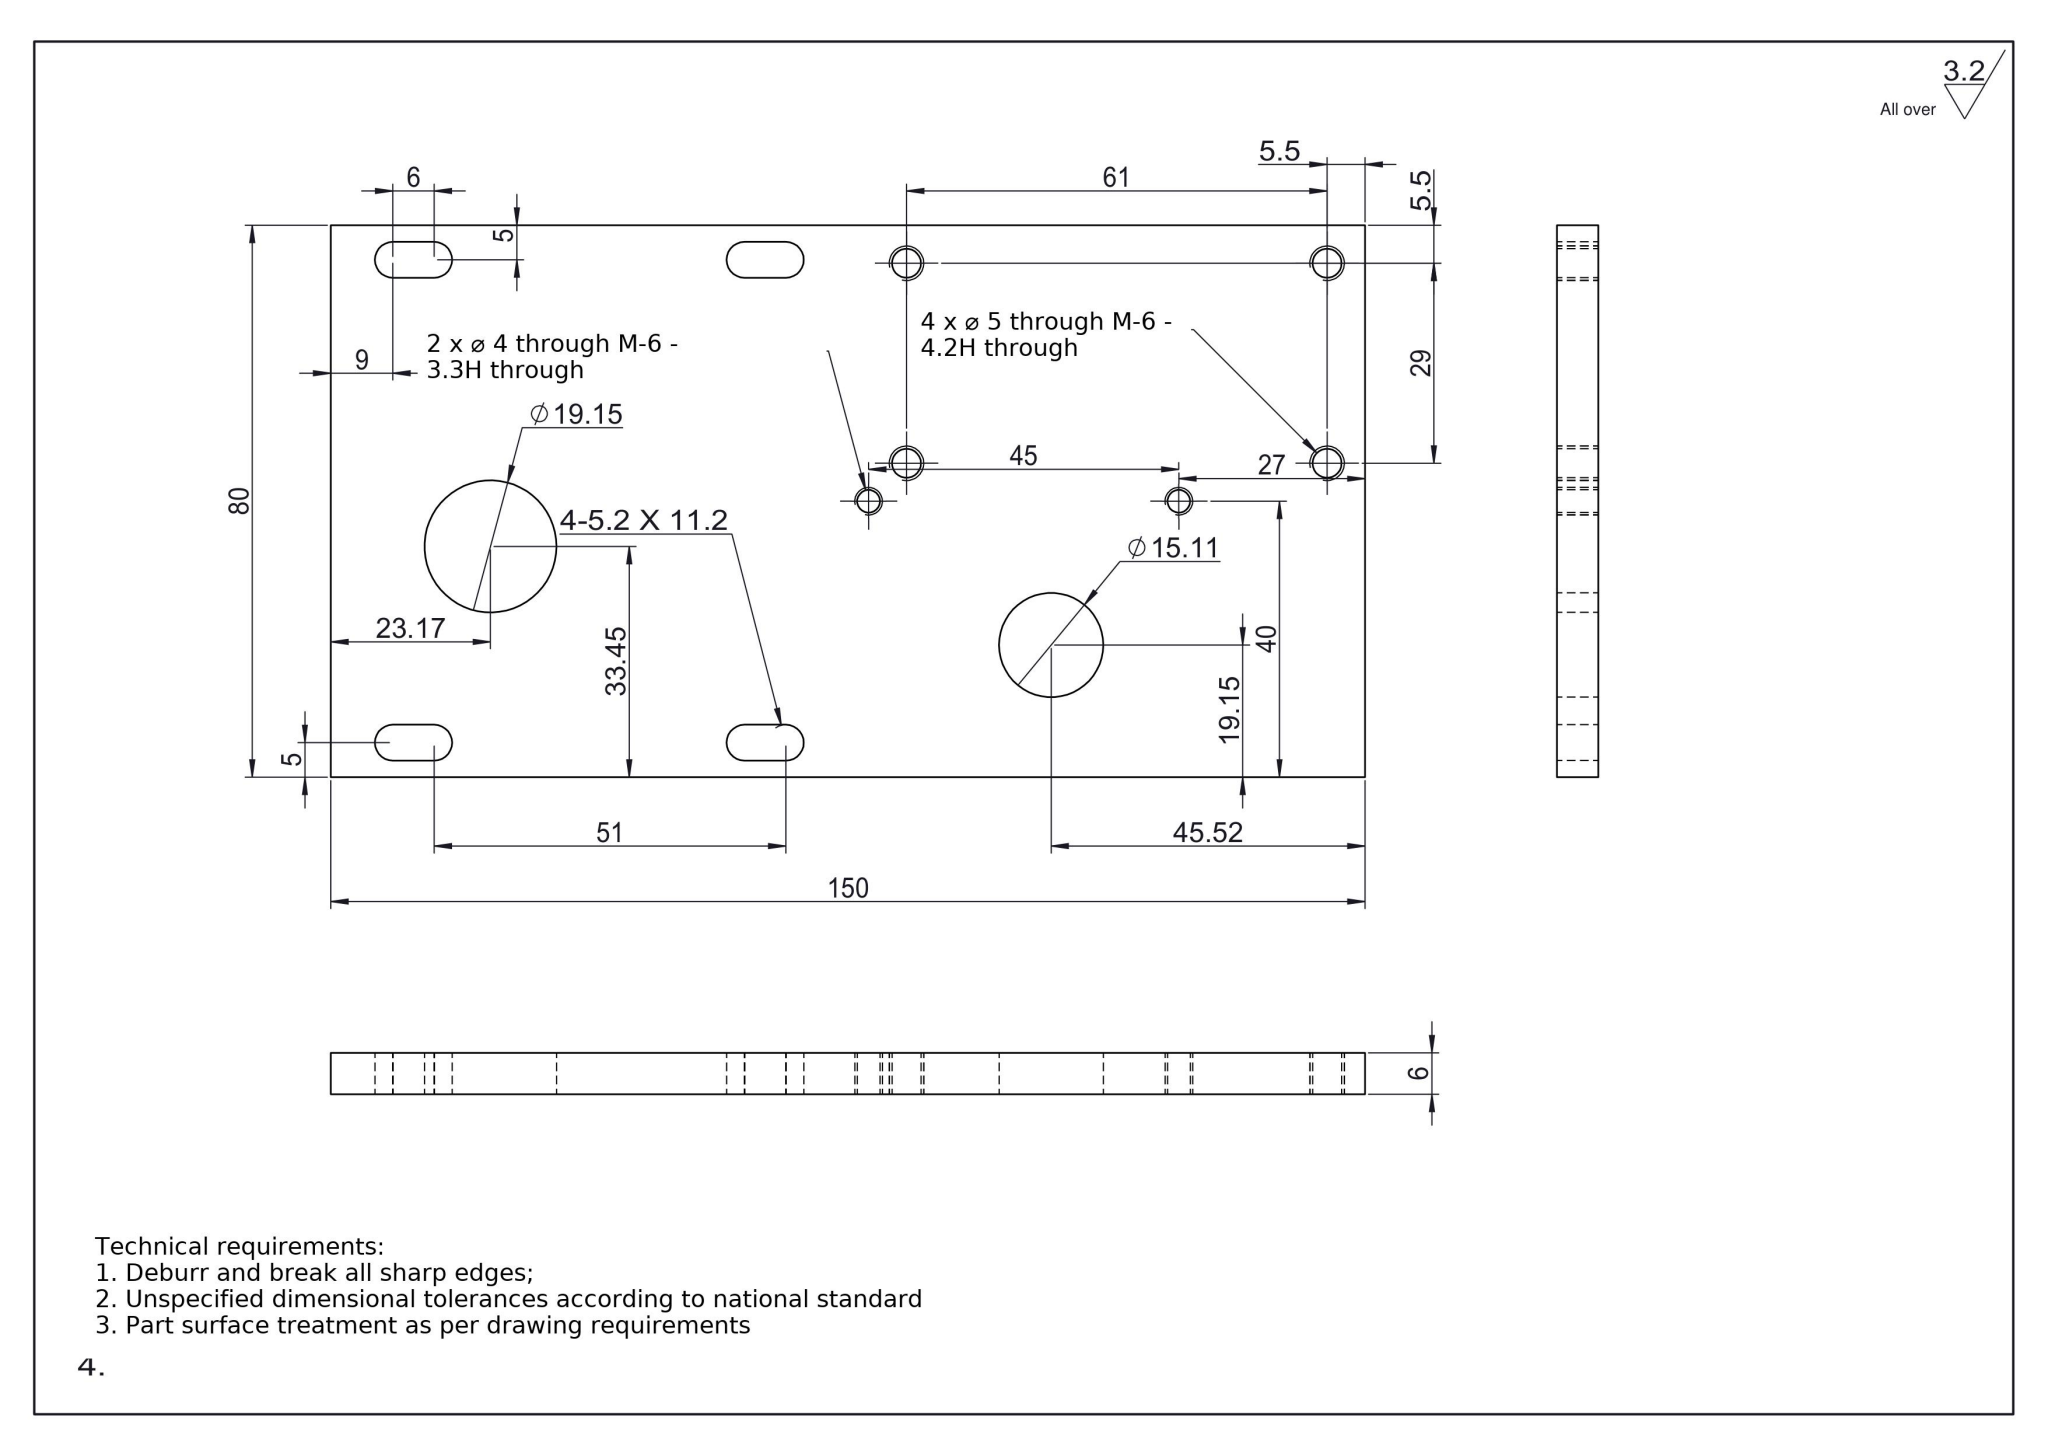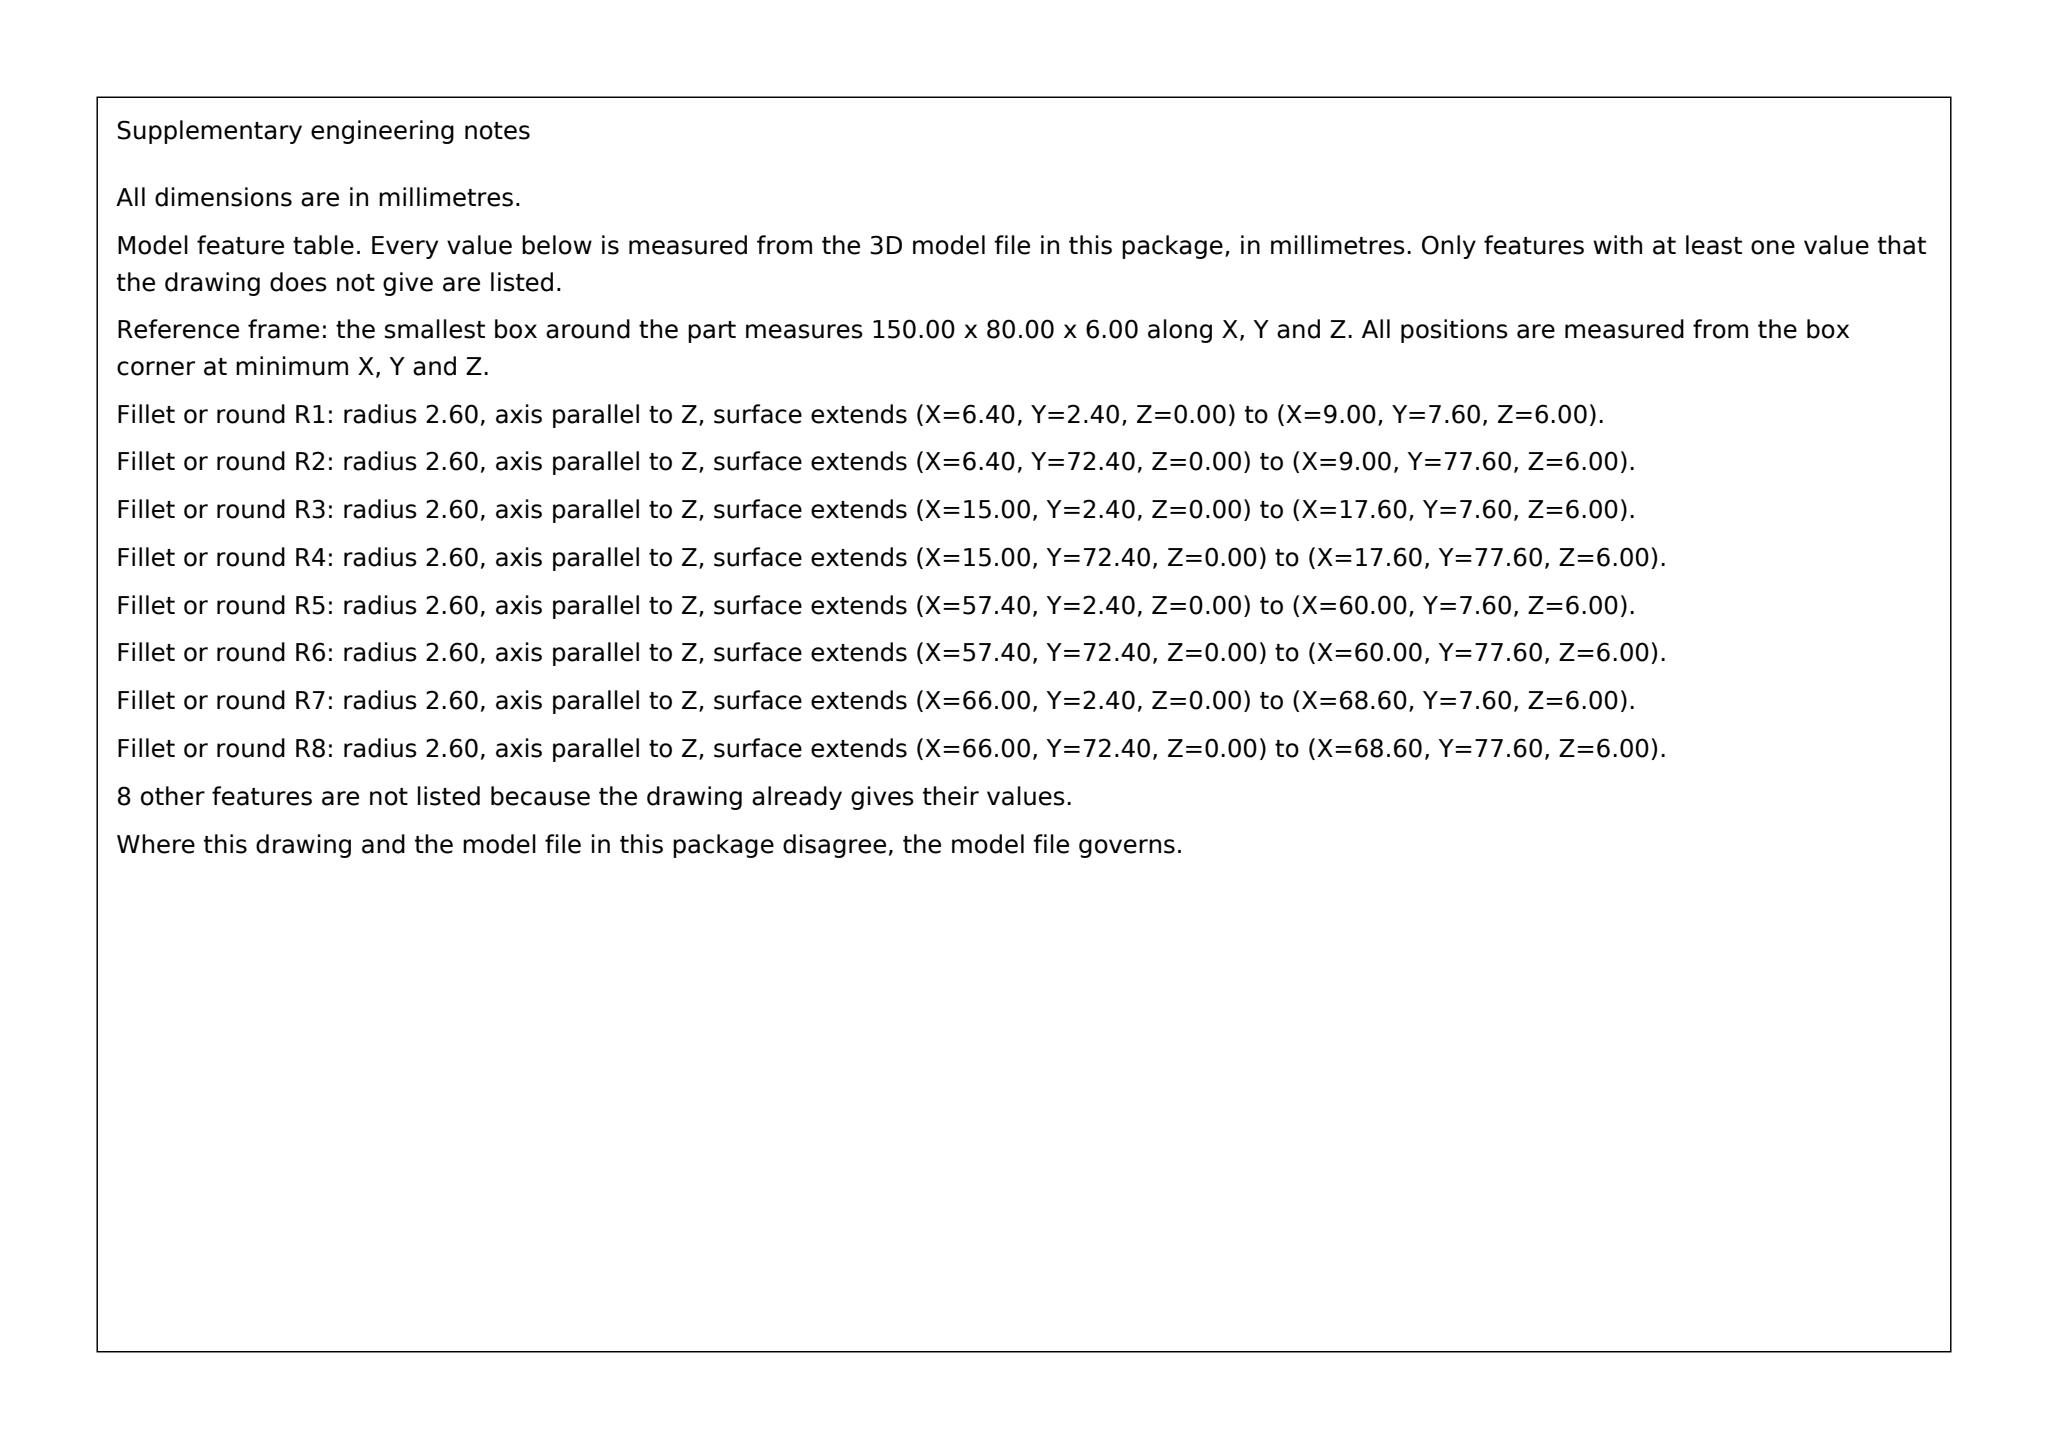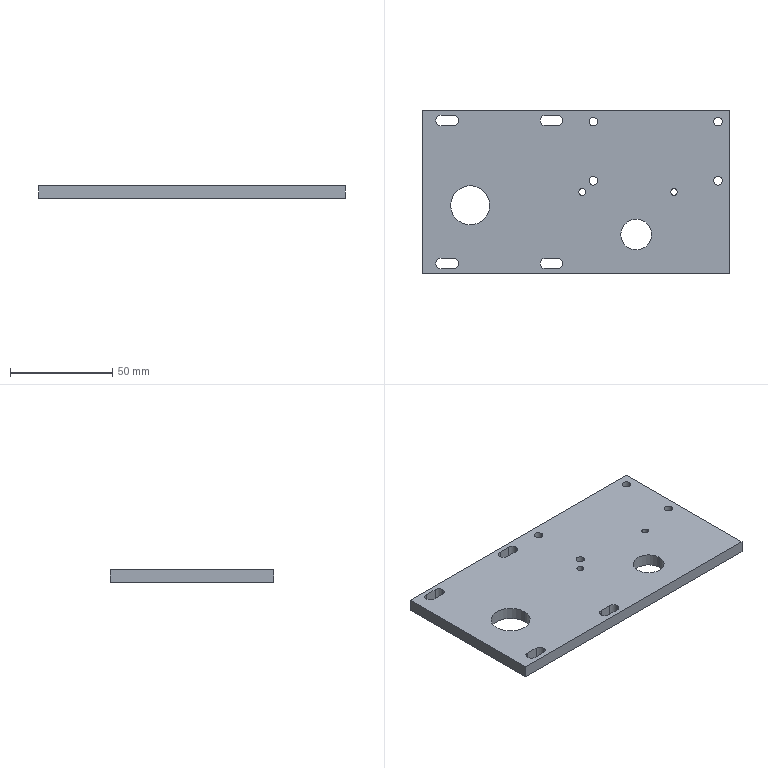Part | SolidWorks | mm | 1 solid | 42 faces | box 150 x 80 x 6 mm | volume 67502 mm3 | cylinder 28 | plane 14 | commonest cylinder face diameters 5.2 x12 4.2 x8 3.3 x4 19.147 x2 15.114 x2
build123d program:
from build123d import *

# Parameters (mm, degrees)
SKETCH1_W           = 150
SKETCH1_H           = 80
BOSS_EXTRUDE1_DEPTH = 6
CUT_EXTRUDE1_DEPTH  = 171.106
M4_TAPPED_HOLE1_D   = 3.3
M5_TAPPED_HOLE1_D   = 4.2
SKETCH7_R           = 9.574
SKETCH7_R_2         = 7.557
CUT_EXTRUDE2_DEPTH  = 80


with BuildPart() as part:
    # Sketch1 → Boss-Extrude1 (new body)
    with BuildSketch(Plane.XY):
        with Locations((75, 40)):
            Rectangle(SKETCH1_W, SKETCH1_H)
    extrude(amount=BOSS_EXTRUDE1_DEPTH)

    # Sketch2 → Cut-Extrude1 (cut, through all)
    with BuildSketch(Plane.XY.offset(6)):
        with BuildLine():
            Line((9, 77.6), (15, 77.6))
            ThreePointArc((15, 77.6), (17.6, 75), (15, 72.4))
            Line((15, 72.4), (9, 72.4))
            ThreePointArc((9, 72.4), (6.4, 75), (9, 77.6))
        make_face()
        with BuildLine():
            Line((60, 77.6), (66, 77.6))
            ThreePointArc((66, 77.6), (68.6, 75), (66, 72.4))
            Line((66, 72.4), (60, 72.4))
            ThreePointArc((60, 72.4), (57.4, 75), (60, 77.6))
        make_face()
        with BuildLine():
            Line((9, 7.6), (15, 7.6))
            ThreePointArc((15, 7.6), (17.6, 5), (15, 2.4))
            Line((15, 2.4), (9, 2.4))
            ThreePointArc((9, 2.4), (6.4, 5), (9, 7.6))
        make_face()
        with BuildLine():
            Line((60, 7.6), (66, 7.6))
            ThreePointArc((66, 7.6), (68.6, 5), (66, 2.4))
            Line((66, 2.4), (60, 2.4))
            ThreePointArc((60, 2.4), (57.4, 5), (60, 7.6))
        make_face()
    extrude(amount=-CUT_EXTRUDE1_DEPTH, mode=Mode.SUBTRACT)

    # M4 Tapped Hole1 (through all)
    with Locations(Plane.XY.offset(6)):
        with Locations((78, 40), (123, 40)):
            Hole(M4_TAPPED_HOLE1_D / 2)

    # M5 Tapped Hole1 (through all)
    with Locations(Plane(origin=(0, 0, 0), x_dir=(-1, 0, 0), z_dir=(0, 0, -1))):
        with Locations((-144.5, 45.5), (-144.5, 74.5), (-83.5, 74.5), (-83.5, 45.5)):
            Hole(M5_TAPPED_HOLE1_D / 2)

    # Sketch7 → Cut-Extrude2 (cut)
    with BuildSketch(Plane.XY.offset(6)):
        with Locations((23.167, 33.453)):
            Circle(SKETCH7_R)
        with Locations((104.484, 19.154)):
            Circle(SKETCH7_R_2)
    extrude(amount=-CUT_EXTRUDE2_DEPTH, mode=Mode.SUBTRACT)


solid = part.part